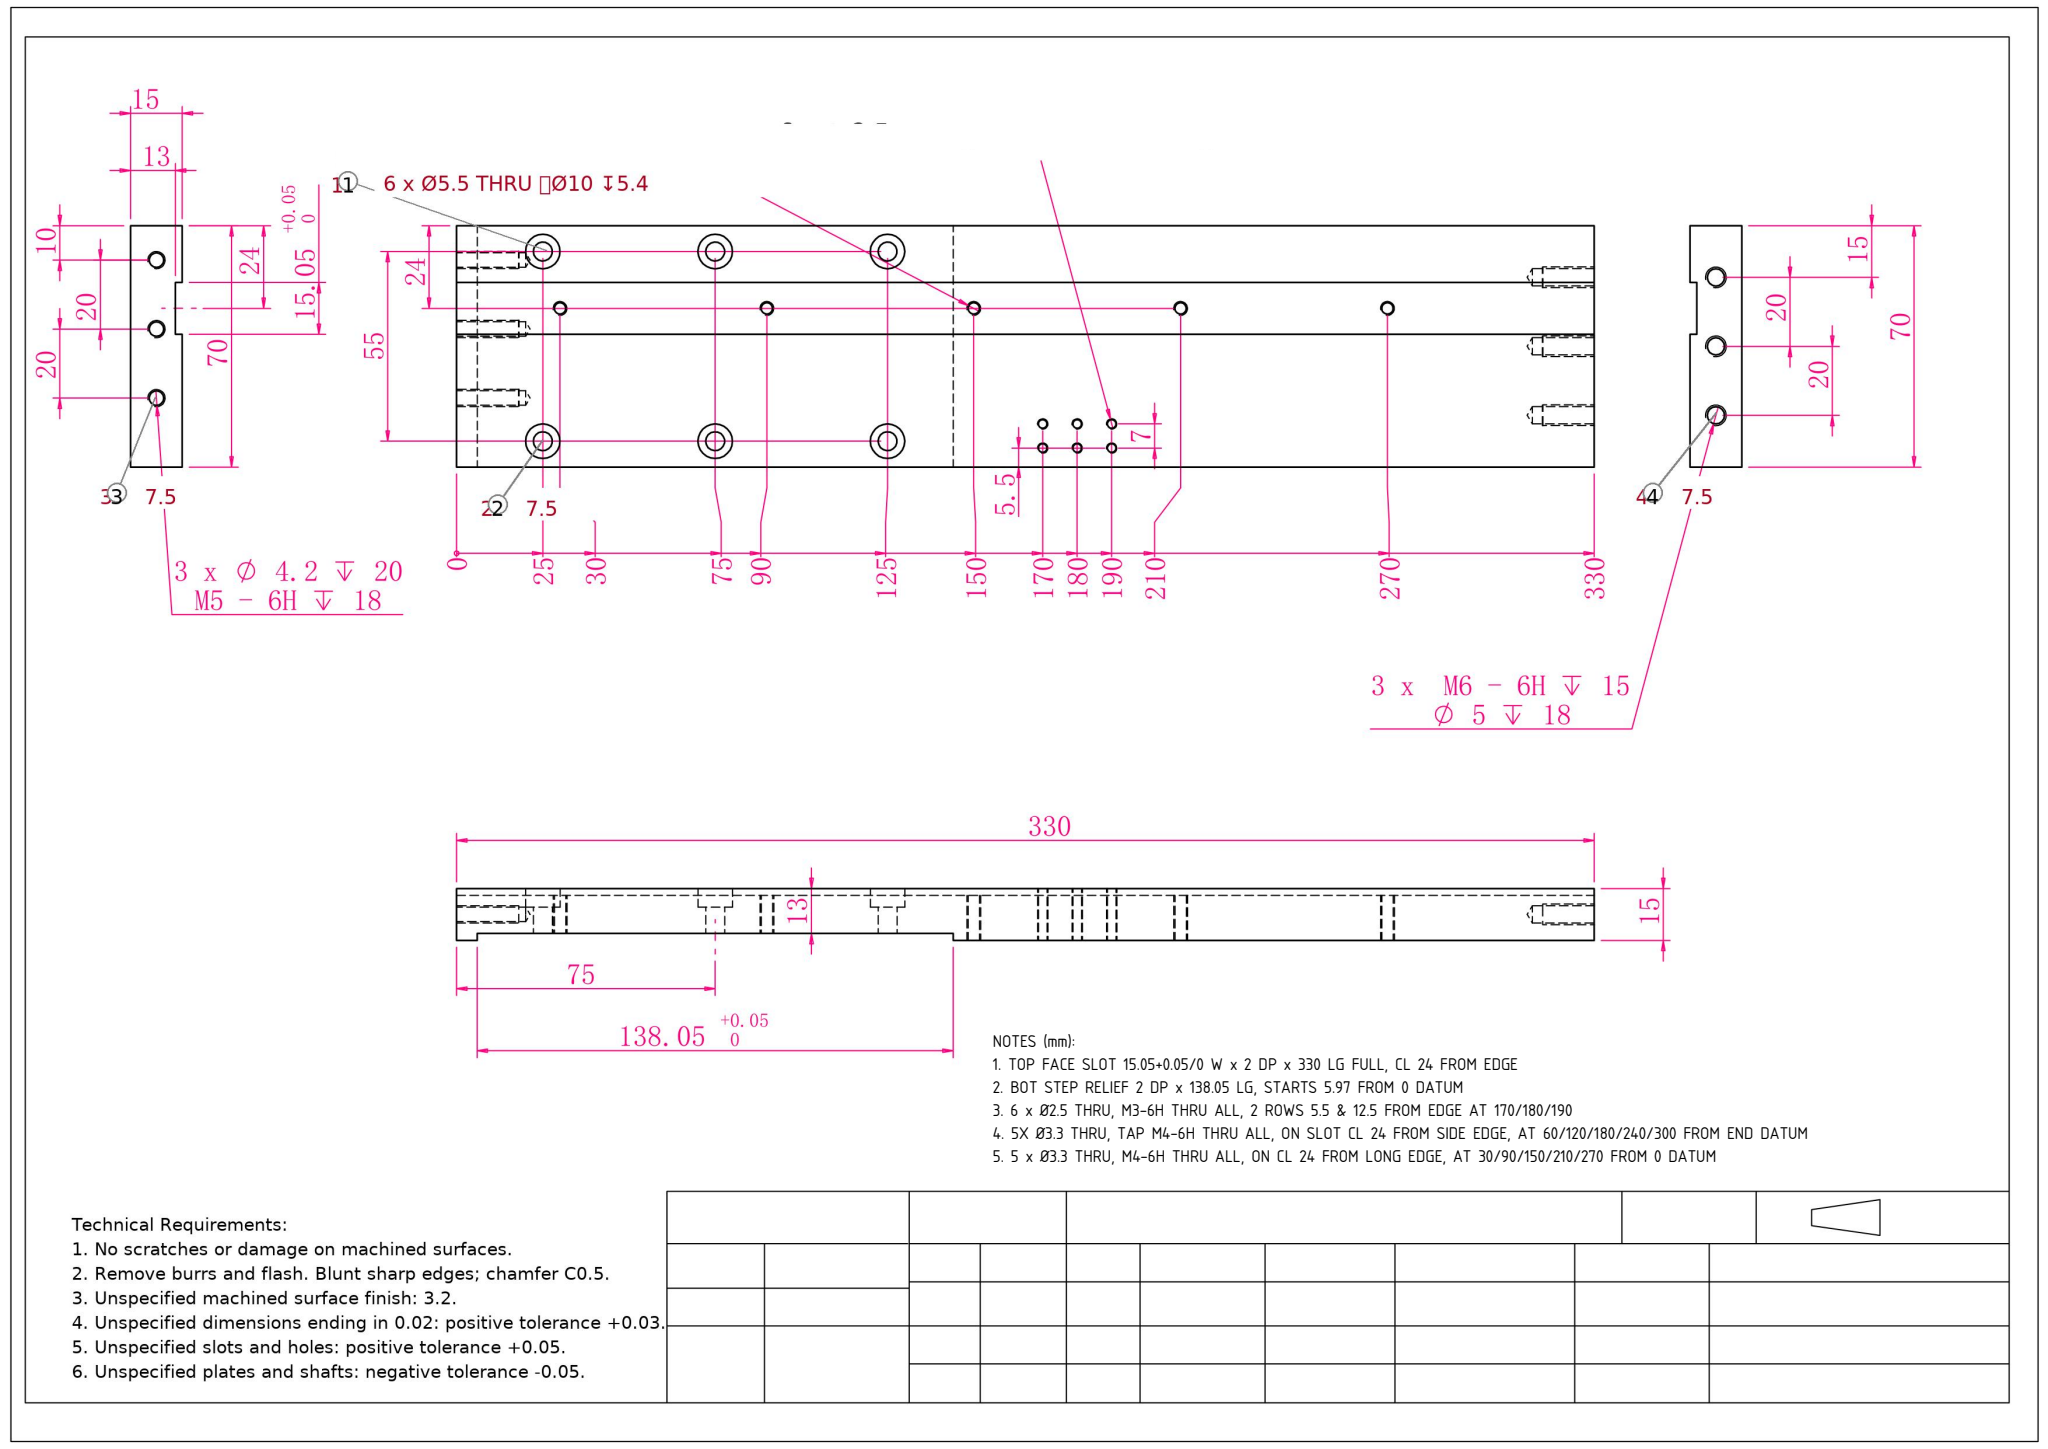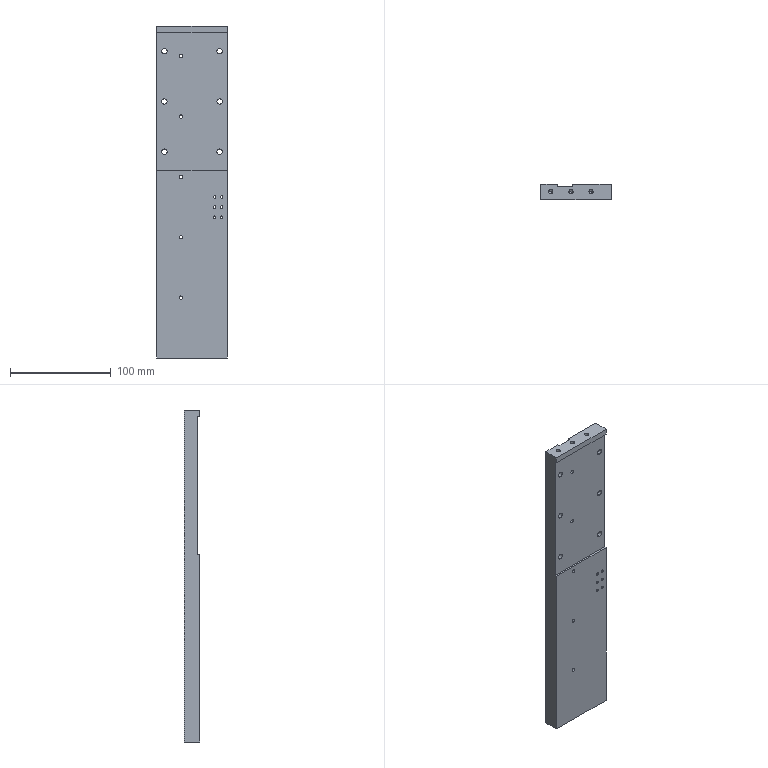Part | SolidWorks | mm | 1 solid | 90 faces | box 70 x 15 x 330 mm | volume 310710 mm3 | cylinder 58 | plane 20 | cone 12 | commonest cylinder face diameters 10 x12 5.5 x12 2.5 x12 3.3 x10 4.2 x6 5 x6
Drawing notes:
TOP FACE SLOT 15.05+0.05/0 W x 2 DP x 330 LG FULL, CL 24 FROM EDGE | from the solid: x-planes 16.48 & 31.53 (W 15.05, CL 24.0 from x=0); y 13.0 vs top 15.0 = 2 DP; runs 330
BOT STEP RELIEF 2 DP x 138.05 LG, STARTS 5.97 FROM 0 DATUM | from the solid: y-plane 2.0 above bottom y=0; z-planes 185.98 & 324.03 = 5.97 & 144.02 from 330 end, span 138.05
6 x Ø2.5 THRU, M3-6H THRU ALL, 2 ROWS 5.5 & 12.5 FROM EDGE AT 170/180/190 | from the solid: Ø2.5 y-axis holes L15.0 full thk at z=140/150/160 (=190/180/170 from datum), x=57.5 & 64.5
5X Ø3.3 THRU, TAP M4-6H THRU ALL, ON SLOT CL 24 FROM SIDE EDGE, AT 60/120/180/240/300 FROM END DATUM | from the solid: cylinders dia 3.3, axis y, pos (x=24, z=60/120/180/240/300), count 5
5 x Ø3.3 THRU, M4-6H THRU ALL, ON CL 24 FROM LONG EDGE, AT 30/90/150/210/270 FROM 0 DATUM | from the solid: cylinders dia 3.3 axis y at x=24.0, z=60/120/180/240/300, length 13/11 through 15 thick plate
build123d program:
from build123d import *

# Parameters (mm, degrees)
SKETCH1_W                                       = 70
SKETCH1_H                                       = 330
EXTRUDE1_DEPTH                                  = 15
SKETCH2_W                                       = 15.05
SKETCH2_H                                       = 330
EXTRUDE2_DEPTH                                  = 2
M6_TAPPED_HOLE1_D                               = 5
M6_TAPPED_HOLE1_DEPTH                           = 18
M6_TAPPED_HOLE1_TIP                             = 1.502
M4_TAPPED_HOLE1_D                               = 3.3
SKETCH45_W                                      = 70
SKETCH45_H                                      = 138.05
CUT_EXTRUDE1_DEPTH                              = 2
M3_TAPPED_HOLE2_D                               = 2.5
M5_TAPPED_HOLE1_D                               = 4.2
M5_TAPPED_HOLE1_DEPTH                           = 20
M5_TAPPED_HOLE1_TIP                             = 1.262
M5_HEX_SOCKET_HEAD_CAP_SCREW_CBORE1_D           = 5.5
M5_HEX_SOCKET_HEAD_CAP_SCREW_CBORE1_CBORE_D     = 10
M5_HEX_SOCKET_HEAD_CAP_SCREW_CBORE1_CBORE_DEPTH = 5.4


with BuildPart() as part:
    # Sketch1 → Extrude1 (new body)
    with BuildSketch(Plane(origin=(0, 0, 0), x_dir=(1, 0, 0), z_dir=(0, 1, 0))):
        with Locations((35, 165)):
            Rectangle(SKETCH1_W, SKETCH1_H)
    extrude(amount=EXTRUDE1_DEPTH)

    # Sketch2 → Extrude2 (cut)
    with BuildSketch(Plane(origin=(0, 15, 0), x_dir=(1, 0, 0), z_dir=(0, 1, 0))):
        with Locations((24, 165)):
            Rectangle(SKETCH2_W, SKETCH2_H)
    extrude(amount=-EXTRUDE2_DEPTH, mode=Mode.SUBTRACT)

    # M6 Tapped Hole1
    with Locations(Plane(origin=(0, 0, -330), x_dir=(-1, 0, 0), z_dir=(0, 0, -1))):
        with Locations((-15, 7.5), (-35, 7.5), (-55, 7.5)):
            Hole(M6_TAPPED_HOLE1_D / 2, depth=M6_TAPPED_HOLE1_DEPTH)
            with Locations((0, 0, -(M6_TAPPED_HOLE1_DEPTH + M6_TAPPED_HOLE1_TIP / 2))):  # 118° drill point
                Cone(0, M6_TAPPED_HOLE1_D / 2, M6_TAPPED_HOLE1_TIP, mode=Mode.SUBTRACT)

    # M4 Tapped Hole1 (through all)
    with Locations(Plane(origin=(0, 15, 0), x_dir=(1, 0, 0), z_dir=(0, 1, 0))):
        with Locations((24, 30), (24, 90), (24, 150), (24, 210), (24, 270)):
            Hole(M4_TAPPED_HOLE1_D / 2)

    # Sketch45 → Cut-Extrude1 (cut)
    with BuildSketch(Plane.XZ):
        with Locations((35, -75)):
            Rectangle(SKETCH45_W, SKETCH45_H)
    extrude(amount=-CUT_EXTRUDE1_DEPTH, mode=Mode.SUBTRACT)

    # M3 Tapped Hole2 (through all)
    with Locations(Plane(origin=(0, 15, 0), x_dir=(1, 0, 0), z_dir=(0, 1, 0))):
        with Locations((57.5, 190), (64.5, 190), (57.5, 180), (64.5, 180), (57.5, 170), (64.5, 170)):
            Hole(M3_TAPPED_HOLE2_D / 2)

    # M5 Tapped Hole1
    with Locations(Plane.XY):
        with Locations((10, 7.5), (30, 7.5), (50, 7.5)):
            Hole(M5_TAPPED_HOLE1_D / 2, depth=M5_TAPPED_HOLE1_DEPTH)
            with Locations((0, 0, -(M5_TAPPED_HOLE1_DEPTH + M5_TAPPED_HOLE1_TIP / 2))):  # 118° drill point
                Cone(0, M5_TAPPED_HOLE1_D / 2, M5_TAPPED_HOLE1_TIP, mode=Mode.SUBTRACT)

    # M5 Hex Socket Head Cap Screw CBORE1 (through all)
    with Locations(Plane(origin=(0, 15, 0), x_dir=(1, 0, 0), z_dir=(0, 1, 0))):
        with Locations((7.5, 125), (7.5, 75), (7.5, 25), (62.5, 25), (62.5, 75), (62.5, 125)):
            CounterBoreHole(M5_HEX_SOCKET_HEAD_CAP_SCREW_CBORE1_D / 2, M5_HEX_SOCKET_HEAD_CAP_SCREW_CBORE1_CBORE_D / 2, M5_HEX_SOCKET_HEAD_CAP_SCREW_CBORE1_CBORE_DEPTH)


solid = part.part